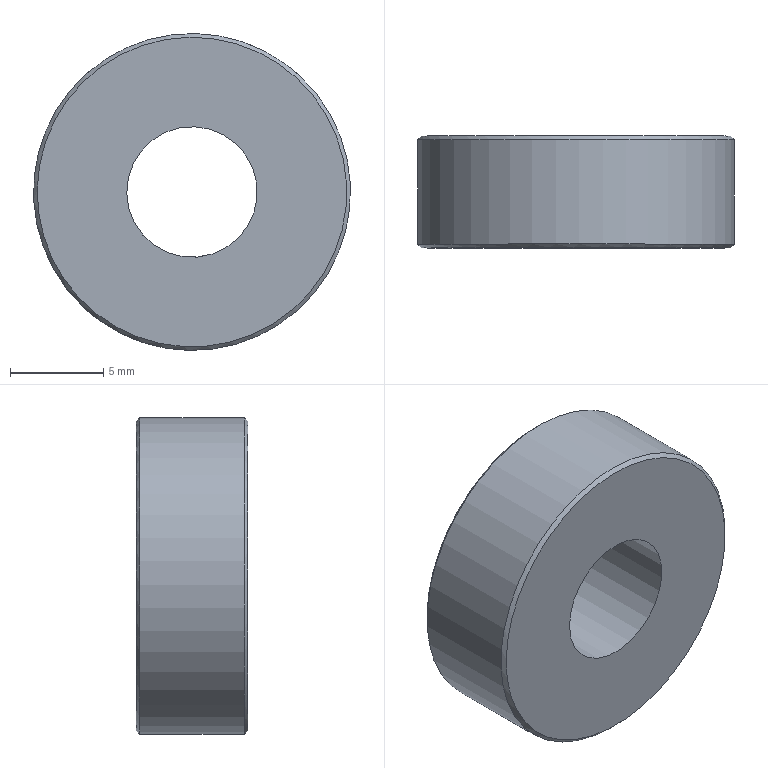Component | NX | TAO_2 | 1 solid | 6 faces | volume 1129 mm3 | cylinder 2 | plane 2 | cone 2 | commonest cylinder face diameters 17 x1 7 x1